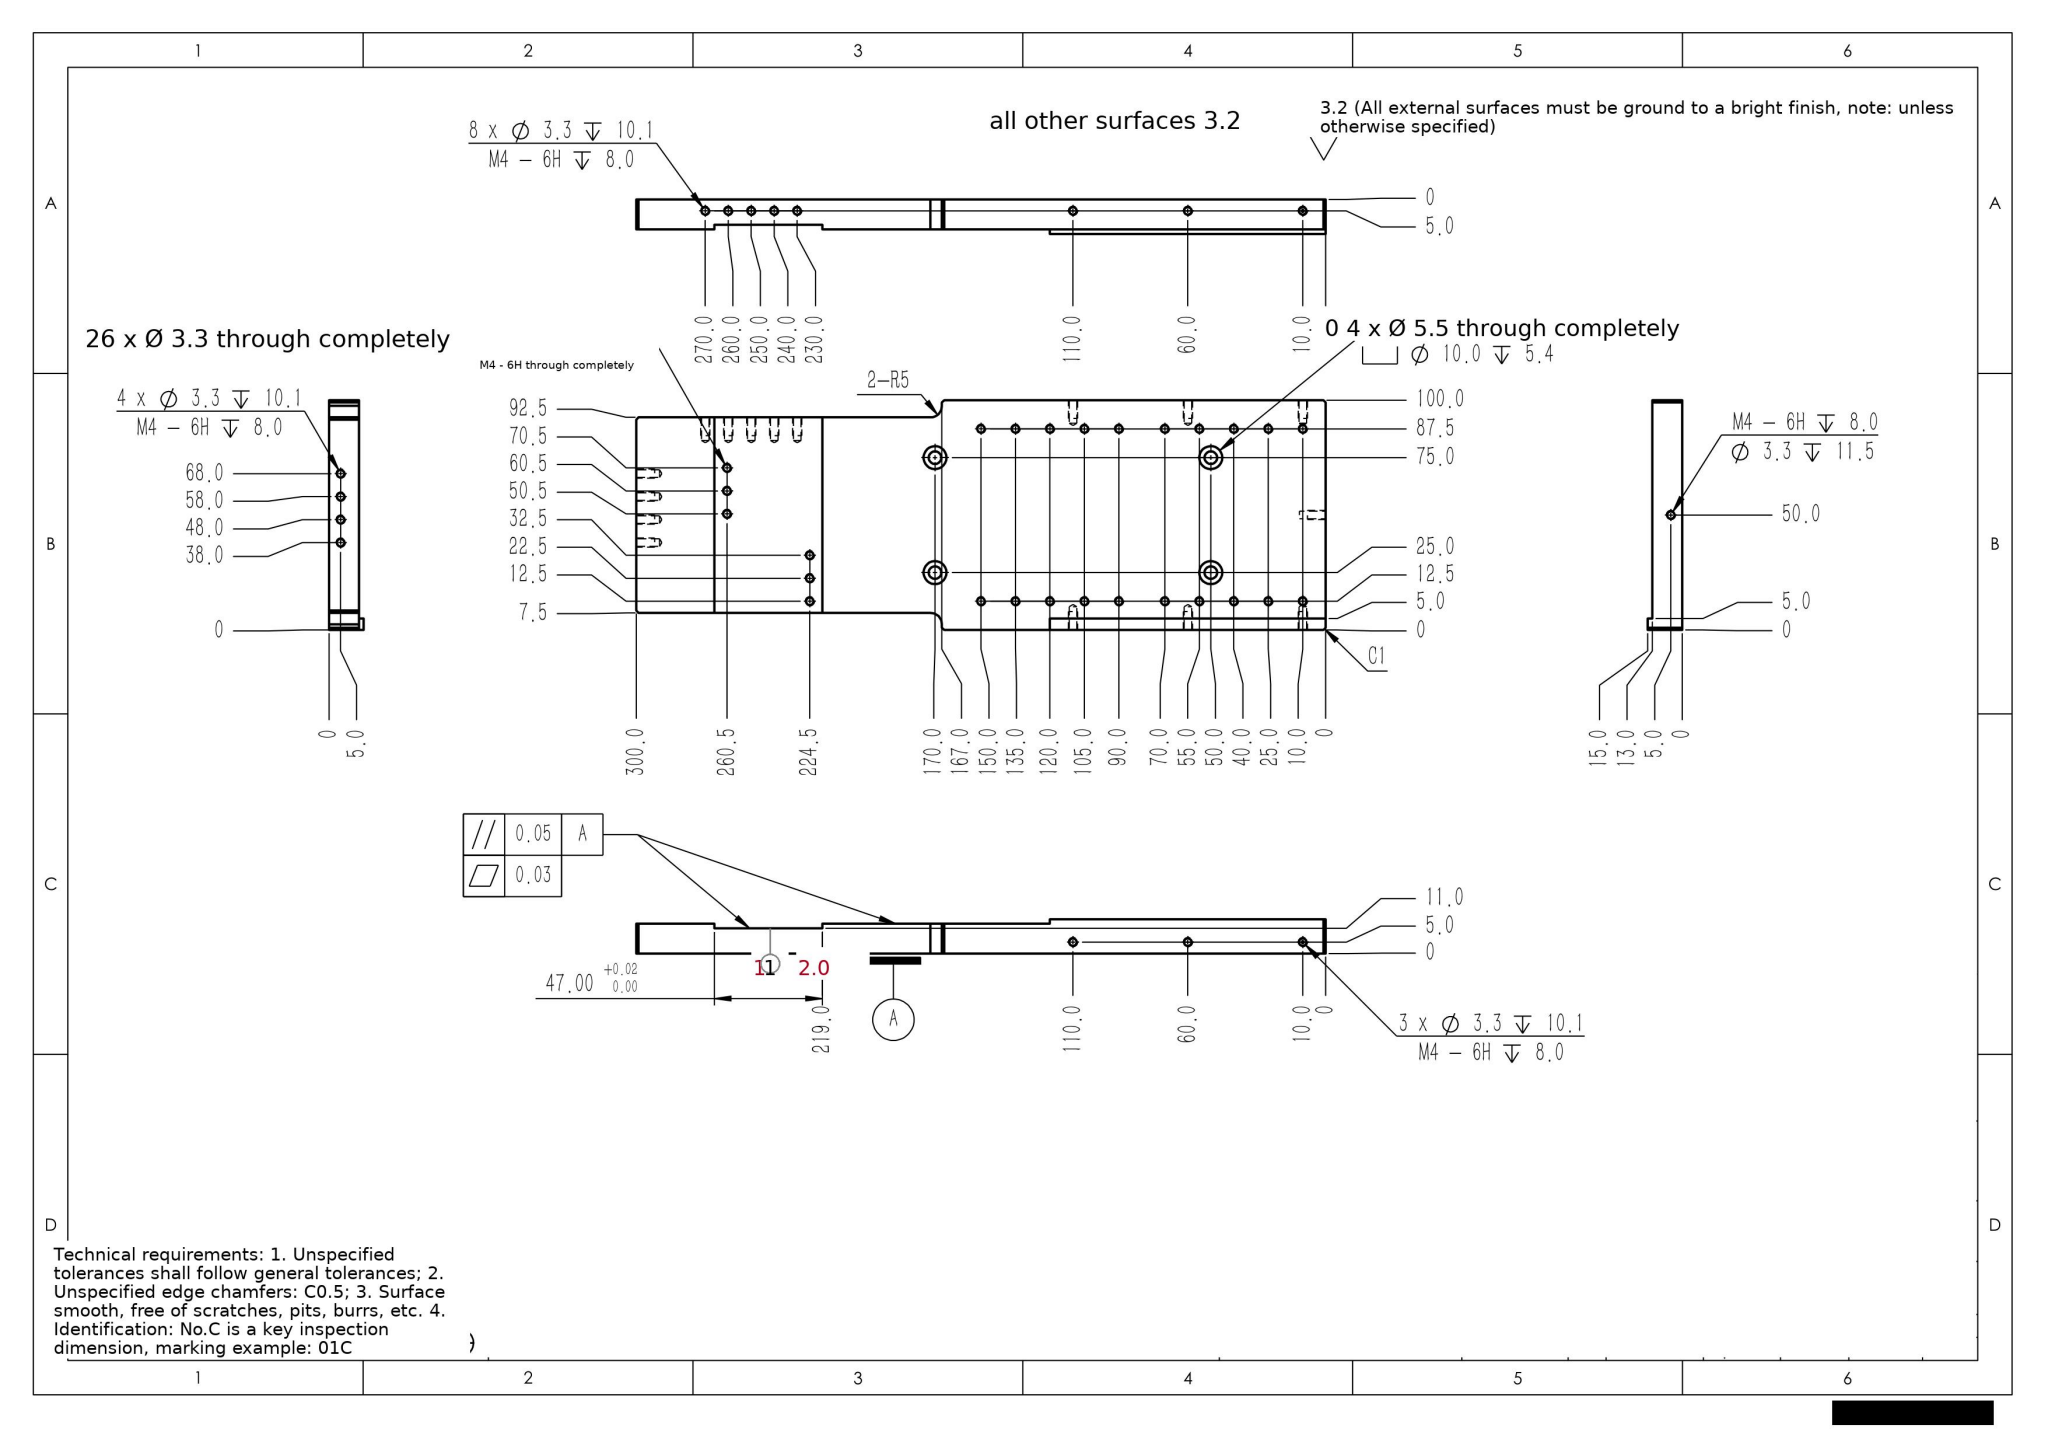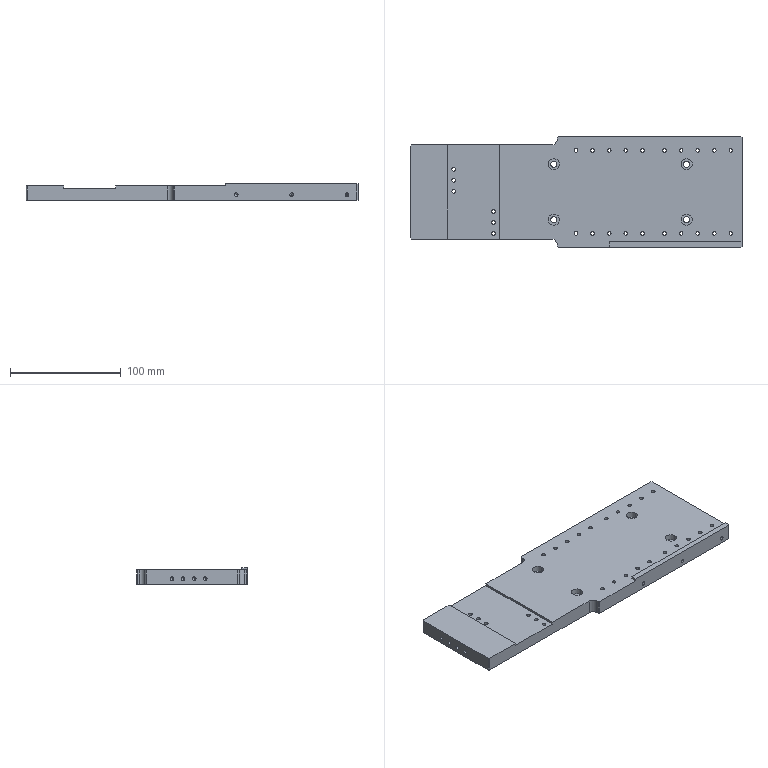Part | SolidWorks | mm | 1 solid | 160 faces | box 300 x 100 x 15 mm | volume 350731 mm3 | cylinder 102 | cone 30 | plane 28 | commonest cylinder face diameters 3.3 x84 10 x10 5.5 x8
build123d program:
from build123d import *

# Parameters (mm, degrees)
SKETCH1_W                                       = 300
SKETCH1_H                                       = 100
BOSS_EXTRUDE1_DEPTH                             = 15
SKETCH2_W                                       = 300
SKETCH2_H                                       = 95
CUT_EXTRUDE1_DEPTH                              = 2
SKETCH3_W                                       = 180
SKETCH3_H                                       = 5
CUT_EXTRUDE5_DEPTH                              = 2
SKETCH4_W                                       = 47
SKETCH4_H                                       = 100
CUT_EXTRUDE6_DEPTH                              = 2
SKETCH5_W                                       = 133
SKETCH5_H                                       = 7.5
CUT_EXTRUDE7_DEPTH                              = 159.647
M4_TAPPED_HOLE1_D                               = 3.3
LPATTERN1_COUNT                                 = 5
LPATTERN1_PITCH                                 = 15
M4_TAPPED_HOLE2_D                               = 3.3
LPATTERN2_COUNT                                 = 3
LPATTERN2_PITCH                                 = 10
LPATTERN3_COUNT                                 = 4
LPATTERN3_PITCH                                 = 10
LPATTERN4_COUNT                                 = 5
LPATTERN4_PITCH                                 = 10
M5_HEX_SOCKET_HEAD_CAP_SCREW_CBORE1_D           = 5.5
M5_HEX_SOCKET_HEAD_CAP_SCREW_CBORE1_CBORE_D     = 10
M5_HEX_SOCKET_HEAD_CAP_SCREW_CBORE1_CBORE_DEPTH = 5.4
M4_TAPPED_HOLE5_D                               = 3.3
M4_TAPPED_HOLE5_DEPTH                           = 10.1
M4_TAPPED_HOLE5_TIP                             = 0.9914
M4_TAPPED_HOLE6_D                               = 3.3
M4_TAPPED_HOLE6_DEPTH                           = 10.1
M4_TAPPED_HOLE6_TIP                             = 0.9914
M4_TAPPED_HOLE7_D                               = 3.3
M4_TAPPED_HOLE7_DEPTH                           = 11.5
CHAMFER1_SIZE                                   = 1
FILLET1_R                                       = 5


with BuildPart() as part:
    # Sketch1 → Boss-Extrude1 (new body)
    with BuildSketch(Plane.XY):
        Rectangle(SKETCH1_W, SKETCH1_H)
    extrude(amount=BOSS_EXTRUDE1_DEPTH)

    # Sketch2 → Cut-Extrude1 (cut)
    with BuildSketch(Plane.XY.offset(15)):
        with Locations((0, 2.5)):
            Rectangle(SKETCH2_W, SKETCH2_H)
    extrude(amount=-CUT_EXTRUDE1_DEPTH, mode=Mode.SUBTRACT)

    # Sketch3 → Cut-Extrude5 (cut)
    with BuildSketch(Plane.XY.offset(13)):
        with Locations((-60, -47.5)):
            Rectangle(SKETCH3_W, SKETCH3_H)
    extrude(amount=CUT_EXTRUDE5_DEPTH, mode=Mode.SUBTRACT)

    # Sketch4 → Cut-Extrude6 (cut)
    with BuildSketch(Plane.XY.offset(13)):
        with Locations((-92.5, 0)):
            Rectangle(SKETCH4_W, SKETCH4_H)
    extrude(amount=-CUT_EXTRUDE6_DEPTH, mode=Mode.SUBTRACT)

    # Sketch5 → Cut-Extrude7 (cut, through all)
    with BuildSketch(Plane.XY.offset(13)):
        with Locations((-83.5, -46.25)):
            Rectangle(SKETCH5_W, SKETCH5_H)
        with Locations((-83.5, 46.25)):
            Rectangle(SKETCH5_W, SKETCH5_H)
    extrude(amount=-CUT_EXTRUDE7_DEPTH, mode=Mode.SUBTRACT)

    # M4 Tapped Hole1 (through all)
    with Locations(Plane.XY.offset(13)):
        with Locations((140, 37.5), (140, -37.5), (60, 37.5), (60, -37.5)):
            m4_tapped_hole1 = Hole(M4_TAPPED_HOLE1_D / 2)

    # LPattern1: M4 Tapped Hole1 ×5
    with Locations(*[(-i * LPATTERN1_PITCH, 0, 0) for i in range(1, LPATTERN1_COUNT)]):
        add(m4_tapped_hole1, mode=Mode.SUBTRACT)

    # M4 Tapped Hole2 (through all)
    with Locations(Plane.XY.offset(11)):
        with Locations((-74.5, -37.5), (-110.5, 0.5)):
            m4_tapped_hole2 = Hole(M4_TAPPED_HOLE2_D / 2)

    # LPattern2: M4 Tapped Hole2 ×3
    with Locations(*[(0, i * LPATTERN2_PITCH, 0) for i in range(1, LPATTERN2_COUNT)]):
        add(m4_tapped_hole2, mode=Mode.SUBTRACT)

    # Sketch12 → M4 Tapped Hole3 (revolve, cut)
    with BuildSketch(Plane(origin=(-150, 18, 5), x_dir=(0, 0, 1), z_dir=(0, 1, 0))):
        Polygon((0, 0), (0, 11.091), (1.65, 10.1), (1.65, 0), align=None)
    m4_tapped_hole3 = revolve(axis=Axis((-156.35, 18, 5), (1, 0, 0)), mode=Mode.SUBTRACT)

    # LPattern3: M4 Tapped Hole3 ×4
    with Locations(*[(0, -i * LPATTERN3_PITCH, 0) for i in range(1, LPATTERN3_COUNT)]):
        add(m4_tapped_hole3, mode=Mode.SUBTRACT)

    # Sketch14 → M4 Tapped Hole4 (revolve, cut)
    with BuildSketch(Plane(origin=(-80, 42.5, 5), x_dir=(0, 0, 1), z_dir=(1, 0, 0))):
        Polygon((0, 0), (0, 11.091), (1.65, 10.1), (1.65, 0), align=None)
    m4_tapped_hole4 = revolve(axis=Axis((-80, 48.85, 5), (0, -1, 0)), mode=Mode.SUBTRACT)

    # LPattern4: M4 Tapped Hole4 ×5
    with Locations(*[(-i * LPATTERN4_PITCH, 0, 0) for i in range(1, LPATTERN4_COUNT)]):
        add(m4_tapped_hole4, mode=Mode.SUBTRACT)

    # M5 Hex Socket Head Cap Screw CBORE1 (through all)
    with Locations(Plane(origin=(0, 0, 13), x_dir=(-1, 0, 0), z_dir=(0, 0, 1))):
        with Locations((-100, -25), (-100, 25), (20, -25), (20, 25)):
            CounterBoreHole(M5_HEX_SOCKET_HEAD_CAP_SCREW_CBORE1_D / 2, M5_HEX_SOCKET_HEAD_CAP_SCREW_CBORE1_CBORE_D / 2, M5_HEX_SOCKET_HEAD_CAP_SCREW_CBORE1_CBORE_DEPTH)

    # M4 Tapped Hole5
    with Locations(Plane(origin=(0, -50, 0), x_dir=(-1, 0, 0), z_dir=(0, -1, 0))):
        with Locations((-140, -5), (-90, -5), (-40, -5)):
            Hole(M4_TAPPED_HOLE5_D / 2, depth=M4_TAPPED_HOLE5_DEPTH)
            with Locations((0, 0, -(M4_TAPPED_HOLE5_DEPTH + M4_TAPPED_HOLE5_TIP / 2))):  # 118° drill point
                Cone(0, M4_TAPPED_HOLE5_D / 2, M4_TAPPED_HOLE5_TIP, mode=Mode.SUBTRACT)

    # M4 Tapped Hole6
    with Locations(Plane(origin=(0, 50, 0), x_dir=(1, 0, 0), z_dir=(0, 1, 0))):
        with Locations((140, -5), (90, -5), (40, -5)):
            Hole(M4_TAPPED_HOLE6_D / 2, depth=M4_TAPPED_HOLE6_DEPTH)
            with Locations((0, 0, -(M4_TAPPED_HOLE6_DEPTH + M4_TAPPED_HOLE6_TIP / 2))):  # 118° drill point
                Cone(0, M4_TAPPED_HOLE6_D / 2, M4_TAPPED_HOLE6_TIP, mode=Mode.SUBTRACT)

    # M4 Tapped Hole7
    with Locations(Plane(origin=(150, 0, 0), x_dir=(0, 0, -1), z_dir=(1, 0, 0))):
        with Locations((-5, 0)):
            Hole(M4_TAPPED_HOLE7_D / 2, depth=M4_TAPPED_HOLE7_DEPTH)

    # Chamfer1
    chamfer1_edges = [part.edges().sort_by_distance(p)[0] for p in [
        (150, 50, 6.5),
        (-150, -42.5, 6.5),
        (-17, -50, 6.5),
        (150, -50, 7.5),
        (-150, 42.5, 6.5),
        (-17, 50, 6.5),
    ]]
    chamfer(chamfer1_edges, length=CHAMFER1_SIZE)

    # Fillet1
    fillet1_edges = [part.edges().sort_by_distance(p)[0] for p in [
        (-17, -42.5, 6.5),
        (-17, 42.5, 6.5),
    ]]
    fillet(fillet1_edges, radius=FILLET1_R)


solid = part.part